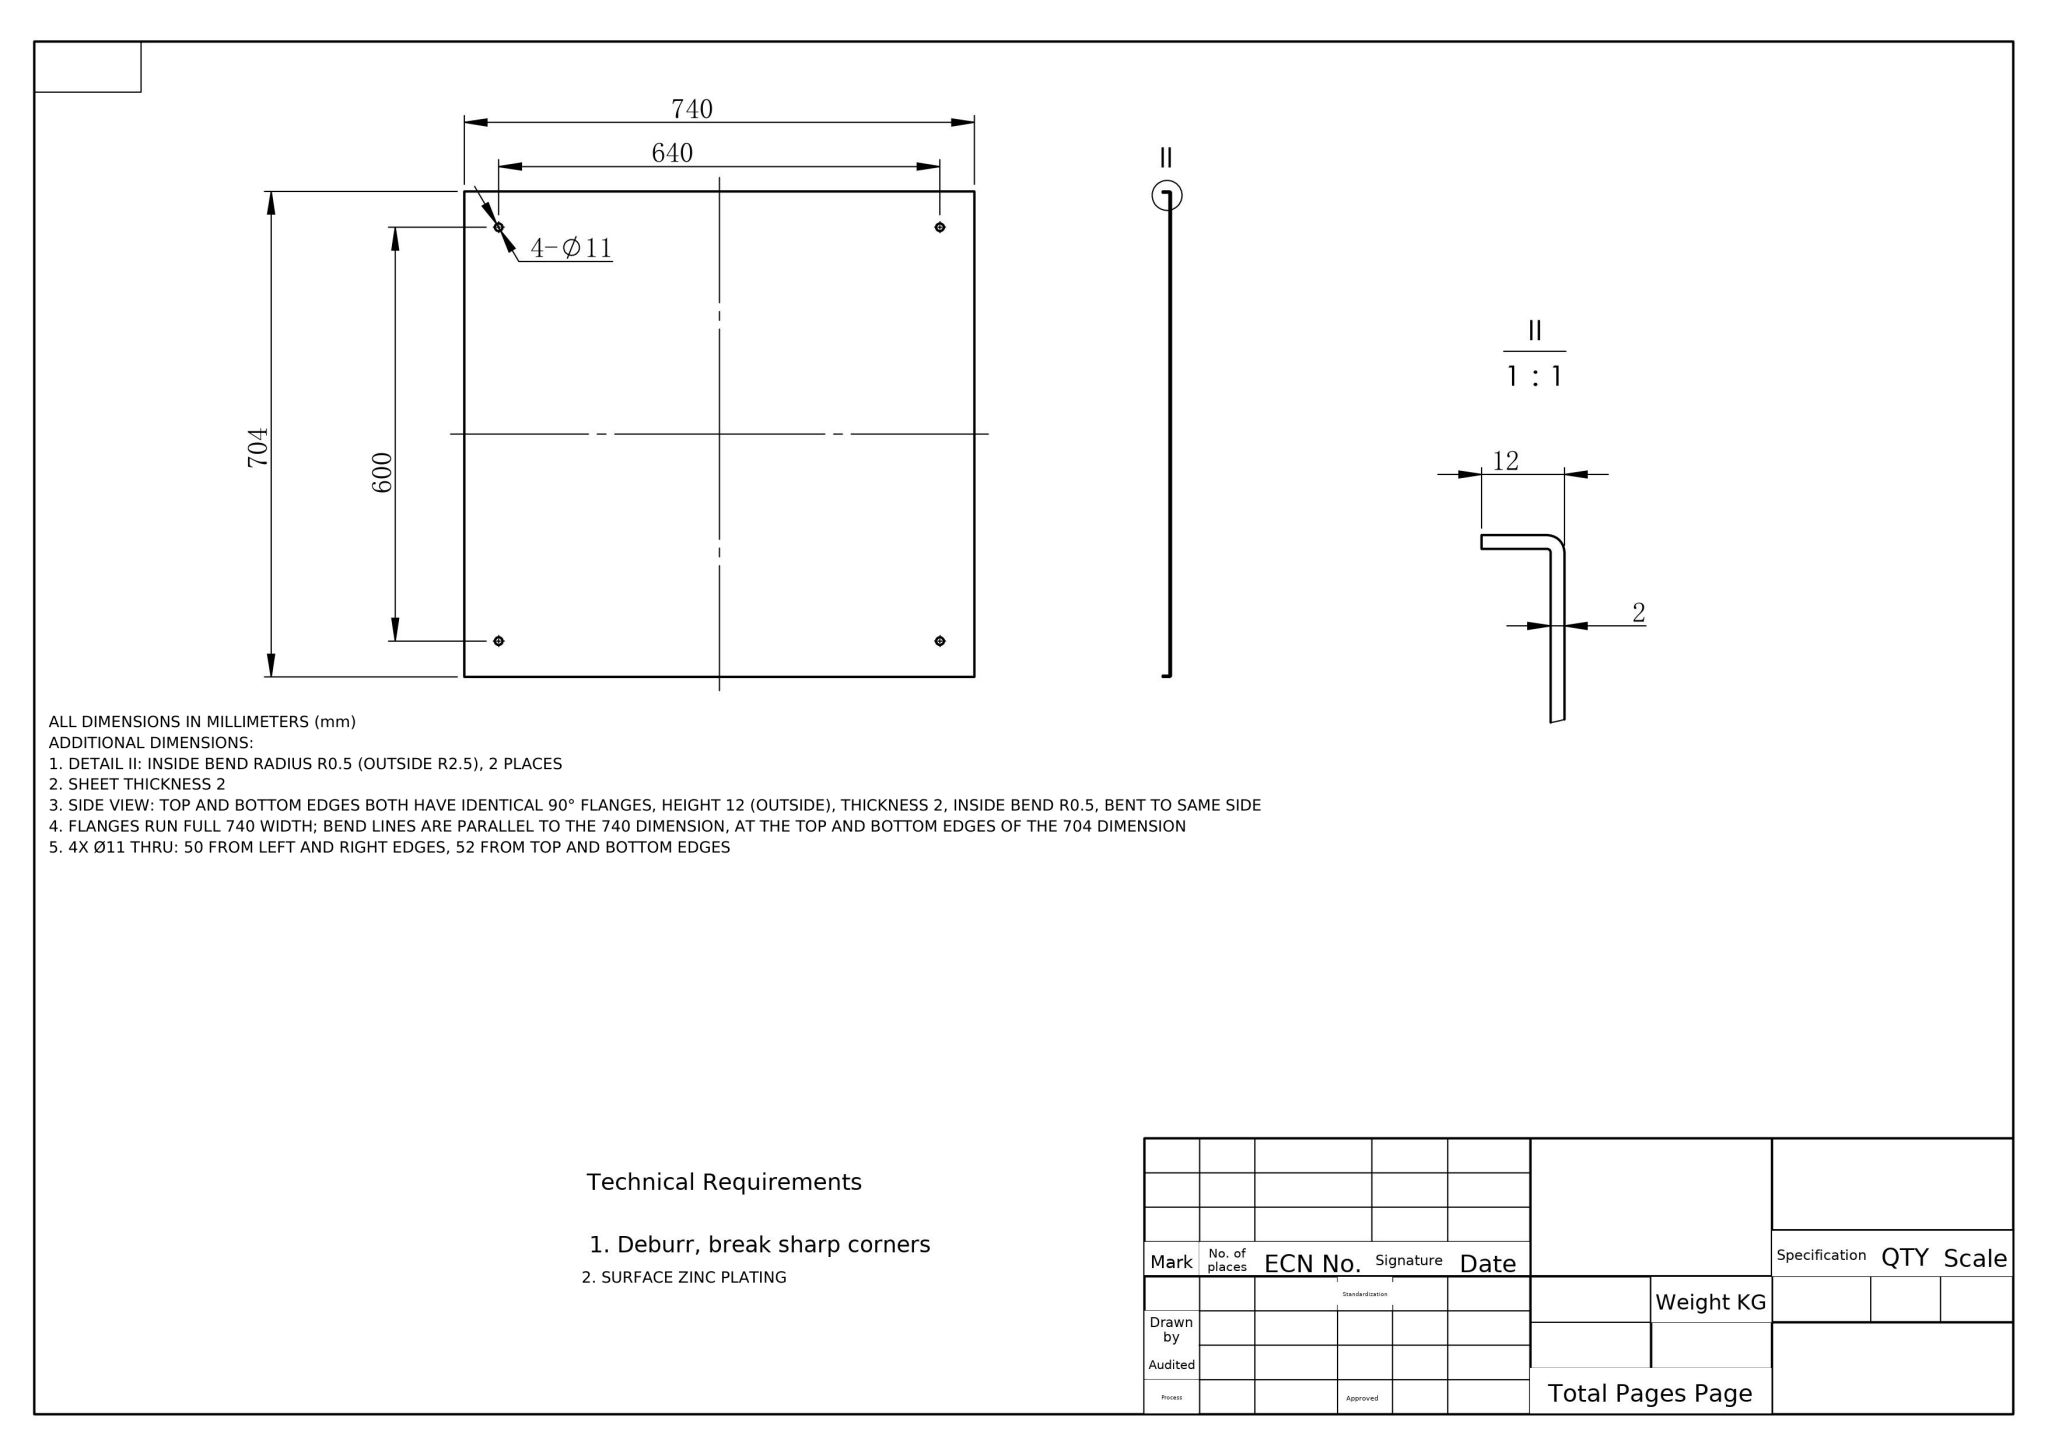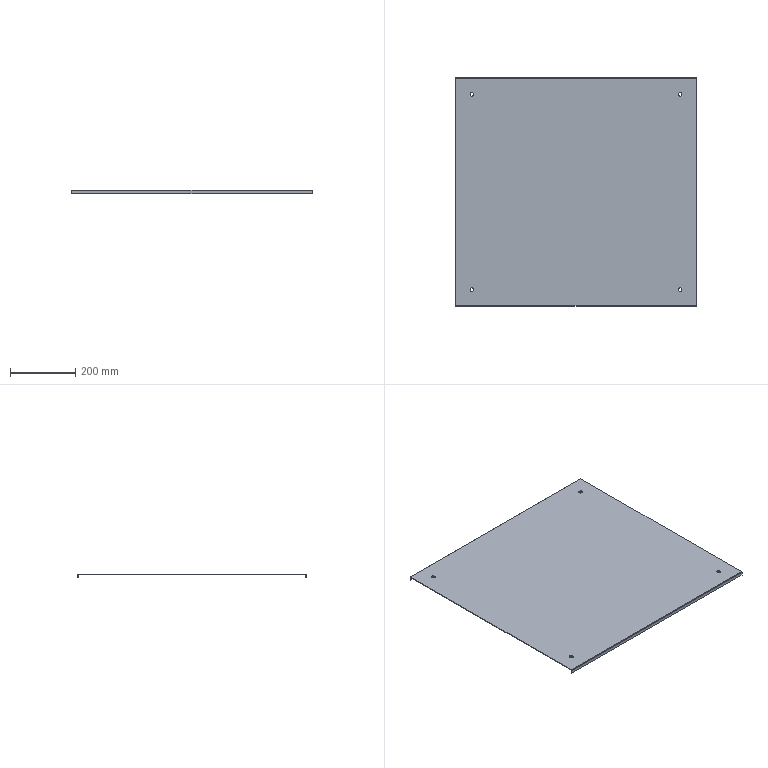Part | NX | mm | 1 solid | 30 faces | box 740 x 704 x 12 mm | volume 1068854 mm3 | plane 18 | cylinder 12 | commonest cylinder face diameters 11 x8 5 x2 1 x2
STEP:
#1=COLOUR_RGB('',0.5294,0.549,0.549);
#2=FILL_AREA_STYLE_COLOUR('',#1);
#3=FILL_AREA_STYLE('',(#2));
#4=SURFACE_STYLE_FILL_AREA(#3);
#5=SURFACE_SIDE_STYLE('',(#4));
#6=SURFACE_STYLE_USAGE(.BOTH.,#5);
#7=PRESENTATION_STYLE_ASSIGNMENT((#6));
#8=CARTESIAN_POINT('',(-305.5,600.,10.));
#9=VERTEX_POINT('',#8);
#10=CARTESIAN_POINT('',(-294.5,600.,10.));
#11=VERTEX_POINT('',#10);
#12=CARTESIAN_POINT('',(-300.,600.,10.));
#13=DIRECTION('',(0.,0.,1.));
#14=DIRECTION('',(1.,0.,0.));
#15=AXIS2_PLACEMENT_3D('',#12,#13,#14);
#16=CIRCLE('',#15,5.5);
#17=EDGE_CURVE('',#9,#11,#16,.T.);
#18=ORIENTED_EDGE('',*,*,#17,.F.);
#19=CARTESIAN_POINT('',(-305.5,600.,12.));
#20=VERTEX_POINT('',#19);
#21=CARTESIAN_POINT('',(-305.5,600.,12.));
#22=DIRECTION('',(0.,0.,1.));
#23=VECTOR('',#22,1000.);
#24=LINE('',#21,#23);
#25=EDGE_CURVE('',#9,#20,#24,.T.);
#26=ORIENTED_EDGE('',*,*,#25,.T.);
#27=CARTESIAN_POINT('',(-294.5,600.,12.));
#28=VERTEX_POINT('',#27);
#29=CARTESIAN_POINT('',(-300.,600.,12.));
#30=DIRECTION('',(0.,0.,1.));
#31=DIRECTION('',(-1.,0.,0.));
#32=AXIS2_PLACEMENT_3D('',#29,#30,#31);
#33=CIRCLE('',#32,5.5);
#34=EDGE_CURVE('',#20,#28,#33,.T.);
#35=ORIENTED_EDGE('',*,*,#34,.T.);
#36=CARTESIAN_POINT('',(-294.5,600.,12.));
#37=DIRECTION('',(0.,0.,1.));
#38=VECTOR('',#37,1000.);
#39=LINE('',#36,#38);
#40=EDGE_CURVE('',#11,#28,#39,.T.);
#41=ORIENTED_EDGE('',*,*,#40,.F.);
#42=EDGE_LOOP('',(#18,#26,#35,#41));
#43=FACE_OUTER_BOUND('',#42,.T.);
#44=CARTESIAN_POINT('',(-300.,600.,12.));
#45=DIRECTION('',(0.,0.,1.));
#46=DIRECTION('',(1.,0.,0.));
#47=AXIS2_PLACEMENT_3D('',#44,#45,#46);
#48=CYLINDRICAL_SURFACE('',#47,5.5);
#49=ADVANCED_FACE('',(#43),#48,.F.);
#50=CARTESIAN_POINT('',(334.5,600.,10.));
#51=VERTEX_POINT('',#50);
#52=CARTESIAN_POINT('',(345.5,600.,10.));
#53=VERTEX_POINT('',#52);
#54=CARTESIAN_POINT('',(340.,600.,10.));
#55=DIRECTION('',(0.,0.,1.));
#56=DIRECTION('',(1.,0.,0.));
#57=AXIS2_PLACEMENT_3D('',#54,#55,#56);
#58=CIRCLE('',#57,5.5);
#59=EDGE_CURVE('',#51,#53,#58,.T.);
#60=ORIENTED_EDGE('',*,*,#59,.F.);
#61=CARTESIAN_POINT('',(334.5,600.,12.));
#62=VERTEX_POINT('',#61);
#63=CARTESIAN_POINT('',(334.5,600.,12.));
#64=DIRECTION('',(0.,0.,1.));
#65=VECTOR('',#64,1000.);
#66=LINE('',#63,#65);
#67=EDGE_CURVE('',#51,#62,#66,.T.);
#68=ORIENTED_EDGE('',*,*,#67,.T.);
#69=CARTESIAN_POINT('',(345.5,600.,12.));
#70=VERTEX_POINT('',#69);
#71=CARTESIAN_POINT('',(340.,600.,12.));
#72=DIRECTION('',(0.,0.,1.));
#73=DIRECTION('',(-1.,0.,0.));
#74=AXIS2_PLACEMENT_3D('',#71,#72,#73);
#75=CIRCLE('',#74,5.5);
#76=EDGE_CURVE('',#62,#70,#75,.T.);
#77=ORIENTED_EDGE('',*,*,#76,.T.);
#78=CARTESIAN_POINT('',(345.5,600.,12.));
#79=DIRECTION('',(0.,0.,1.));
#80=VECTOR('',#79,1000.);
#81=LINE('',#78,#80);
#82=EDGE_CURVE('',#53,#70,#81,.T.);
#83=ORIENTED_EDGE('',*,*,#82,.F.);
#84=EDGE_LOOP('',(#60,#68,#77,#83));
#85=FACE_OUTER_BOUND('',#84,.T.);
#86=CARTESIAN_POINT('',(340.,600.,12.));
#87=DIRECTION('',(0.,0.,1.));
#88=DIRECTION('',(1.,0.,0.));
#89=AXIS2_PLACEMENT_3D('',#86,#87,#88);
#90=CYLINDRICAL_SURFACE('',#89,5.5);
#91=ADVANCED_FACE('',(#85),#90,.F.);
#92=CARTESIAN_POINT('',(334.5,1200.,10.));
#93=VERTEX_POINT('',#92);
#94=CARTESIAN_POINT('',(345.5,1200.,10.));
#95=VERTEX_POINT('',#94);
#96=CARTESIAN_POINT('',(340.,1200.,10.));
#97=DIRECTION('',(0.,0.,1.));
#98=DIRECTION('',(1.,0.,0.));
#99=AXIS2_PLACEMENT_3D('',#96,#97,#98);
#100=CIRCLE('',#99,5.5);
#101=EDGE_CURVE('',#93,#95,#100,.T.);
#102=ORIENTED_EDGE('',*,*,#101,.F.);
#103=CARTESIAN_POINT('',(334.5,1200.,12.));
#104=VERTEX_POINT('',#103);
#105=CARTESIAN_POINT('',(334.5,1200.,12.));
#106=DIRECTION('',(0.,0.,1.));
#107=VECTOR('',#106,1000.);
#108=LINE('',#105,#107);
#109=EDGE_CURVE('',#93,#104,#108,.T.);
#110=ORIENTED_EDGE('',*,*,#109,.T.);
#111=CARTESIAN_POINT('',(345.5,1200.,12.));
#112=VERTEX_POINT('',#111);
#113=CARTESIAN_POINT('',(340.,1200.,12.));
#114=DIRECTION('',(0.,0.,1.));
#115=DIRECTION('',(1.,0.,0.));
#116=AXIS2_PLACEMENT_3D('',#113,#114,#115);
#117=CIRCLE('',#116,5.5);
#118=EDGE_CURVE('',#104,#112,#117,.T.);
#119=ORIENTED_EDGE('',*,*,#118,.T.);
#120=CARTESIAN_POINT('',(345.5,1200.,12.));
#121=DIRECTION('',(0.,0.,1.));
#122=VECTOR('',#121,1000.);
#123=LINE('',#120,#122);
#124=EDGE_CURVE('',#95,#112,#123,.T.);
#125=ORIENTED_EDGE('',*,*,#124,.F.);
#126=EDGE_LOOP('',(#102,#110,#119,#125));
#127=FACE_OUTER_BOUND('',#126,.T.);
#128=CARTESIAN_POINT('',(340.,1200.,12.));
#129=DIRECTION('',(0.,0.,1.));
#130=DIRECTION('',(1.,0.,0.));
#131=AXIS2_PLACEMENT_3D('',#128,#129,#130);
#132=CYLINDRICAL_SURFACE('',#131,5.5);
#133=ADVANCED_FACE('',(#127),#132,.F.);
#134=CARTESIAN_POINT('',(-305.5,1200.,10.));
#135=VERTEX_POINT('',#134);
#136=CARTESIAN_POINT('',(-294.5,1200.,10.));
#137=VERTEX_POINT('',#136);
#138=CARTESIAN_POINT('',(-300.,1200.,10.));
#139=DIRECTION('',(0.,0.,1.));
#140=DIRECTION('',(1.,0.,0.));
#141=AXIS2_PLACEMENT_3D('',#138,#139,#140);
#142=CIRCLE('',#141,5.5);
#143=EDGE_CURVE('',#135,#137,#142,.T.);
#144=ORIENTED_EDGE('',*,*,#143,.F.);
#145=CARTESIAN_POINT('',(-305.5,1200.,12.));
#146=VERTEX_POINT('',#145);
#147=CARTESIAN_POINT('',(-305.5,1200.,12.));
#148=DIRECTION('',(0.,0.,1.));
#149=VECTOR('',#148,1000.);
#150=LINE('',#147,#149);
#151=EDGE_CURVE('',#135,#146,#150,.T.);
#152=ORIENTED_EDGE('',*,*,#151,.T.);
#153=CARTESIAN_POINT('',(-294.5,1200.,12.));
#154=VERTEX_POINT('',#153);
#155=CARTESIAN_POINT('',(-300.,1200.,12.));
#156=DIRECTION('',(0.,0.,1.));
#157=DIRECTION('',(1.,0.,0.));
#158=AXIS2_PLACEMENT_3D('',#155,#156,#157);
#159=CIRCLE('',#158,5.5);
#160=EDGE_CURVE('',#146,#154,#159,.T.);
#161=ORIENTED_EDGE('',*,*,#160,.T.);
#162=CARTESIAN_POINT('',(-294.5,1200.,12.));
#163=DIRECTION('',(0.,0.,1.));
#164=VECTOR('',#163,1000.);
#165=LINE('',#162,#164);
#166=EDGE_CURVE('',#137,#154,#165,.T.);
#167=ORIENTED_EDGE('',*,*,#166,.F.);
#168=EDGE_LOOP('',(#144,#152,#161,#167));
#169=FACE_OUTER_BOUND('',#168,.T.);
#170=CARTESIAN_POINT('',(-300.,1200.,12.));
#171=DIRECTION('',(0.,0.,1.));
#172=DIRECTION('',(1.,0.,0.));
#173=AXIS2_PLACEMENT_3D('',#170,#171,#172);
#174=CYLINDRICAL_SURFACE('',#173,5.5);
#175=ADVANCED_FACE('',(#169),#174,.F.);
#176=CARTESIAN_POINT('',(-300.,1200.,12.));
#177=DIRECTION('',(0.,0.,1.));
#178=DIRECTION('',(1.,0.,0.));
#179=AXIS2_PLACEMENT_3D('',#176,#177,#178);
#180=CIRCLE('',#179,5.5);
#181=EDGE_CURVE('',#154,#146,#180,.T.);
#182=ORIENTED_EDGE('',*,*,#181,.F.);
#183=ORIENTED_EDGE('',*,*,#160,.F.);
#184=EDGE_LOOP('',(#182,#183));
#185=FACE_BOUND('',#184,.T.);
#186=CARTESIAN_POINT('',(340.,1200.,12.));
#187=DIRECTION('',(0.,0.,1.));
#188=DIRECTION('',(1.,0.,0.));
#189=AXIS2_PLACEMENT_3D('',#186,#187,#188);
#190=CIRCLE('',#189,5.5);
#191=EDGE_CURVE('',#112,#104,#190,.T.);
#192=ORIENTED_EDGE('',*,*,#191,.F.);
#193=ORIENTED_EDGE('',*,*,#118,.F.);
#194=EDGE_LOOP('',(#192,#193));
#195=FACE_BOUND('',#194,.T.);
#196=CARTESIAN_POINT('',(340.,600.,12.));
#197=DIRECTION('',(0.,0.,1.));
#198=DIRECTION('',(-1.,0.,0.));
#199=AXIS2_PLACEMENT_3D('',#196,#197,#198);
#200=CIRCLE('',#199,5.5);
#201=EDGE_CURVE('',#70,#62,#200,.T.);
#202=ORIENTED_EDGE('',*,*,#201,.F.);
#203=ORIENTED_EDGE('',*,*,#76,.F.);
#204=EDGE_LOOP('',(#202,#203));
#205=FACE_BOUND('',#204,.T.);
#206=CARTESIAN_POINT('',(-300.,600.,12.));
#207=DIRECTION('',(0.,0.,1.));
#208=DIRECTION('',(-1.,0.,0.));
#209=AXIS2_PLACEMENT_3D('',#206,#207,#208);
#210=CIRCLE('',#209,5.5);
#211=EDGE_CURVE('',#28,#20,#210,.T.);
#212=ORIENTED_EDGE('',*,*,#211,.F.);
#213=ORIENTED_EDGE('',*,*,#34,.F.);
#214=EDGE_LOOP('',(#212,#213));
#215=FACE_BOUND('',#214,.T.);
#216=CARTESIAN_POINT('',(-350.,550.5,12.));
#217=VERTEX_POINT('',#216);
#218=CARTESIAN_POINT('',(390.,550.5,12.));
#219=VERTEX_POINT('',#218);
#220=CARTESIAN_POINT('',(-350.,550.5,12.));
#221=DIRECTION('',(1.,0.,0.));
#222=VECTOR('',#221,1000.);
#223=LINE('',#220,#222);
#224=EDGE_CURVE('',#217,#219,#223,.T.);
#225=ORIENTED_EDGE('',*,*,#224,.T.);
#226=CARTESIAN_POINT('',(390.,1249.5,12.));
#227=VERTEX_POINT('',#226);
#228=CARTESIAN_POINT('',(390.,550.,12.));
#229=DIRECTION('',(0.,1.,0.));
#230=VECTOR('',#229,1000.);
#231=LINE('',#228,#230);
#232=EDGE_CURVE('',#219,#227,#231,.T.);
#233=ORIENTED_EDGE('',*,*,#232,.T.);
#234=CARTESIAN_POINT('',(-350.,1249.5,12.));
#235=VERTEX_POINT('',#234);
#236=CARTESIAN_POINT('',(390.,1249.5,12.));
#237=DIRECTION('',(-1.,0.,0.));
#238=VECTOR('',#237,1000.);
#239=LINE('',#236,#238);
#240=EDGE_CURVE('',#227,#235,#239,.T.);
#241=ORIENTED_EDGE('',*,*,#240,.T.);
#242=CARTESIAN_POINT('',(-350.,550.,12.));
#243=DIRECTION('',(0.,-1.,0.));
#244=VECTOR('',#243,1000.);
#245=LINE('',#242,#244);
#246=EDGE_CURVE('',#235,#217,#245,.T.);
#247=ORIENTED_EDGE('',*,*,#246,.T.);
#248=EDGE_LOOP('',(#225,#233,#241,#247));
#249=FACE_OUTER_BOUND('',#248,.T.);
#250=CARTESIAN_POINT('',(0.,0.,12.));
#251=DIRECTION('',(0.,0.,-1.));
#252=DIRECTION('',(-1.,0.,0.));
#253=AXIS2_PLACEMENT_3D('',#250,#251,#252);
#254=PLANE('',#253);
#255=ADVANCED_FACE('',(#185,#195,#205,#215,#249),#254,.F.);
#256=CARTESIAN_POINT('',(-300.,1200.,10.));
#257=DIRECTION('',(0.,0.,1.));
#258=DIRECTION('',(1.,0.,0.));
#259=AXIS2_PLACEMENT_3D('',#256,#257,#258);
#260=CIRCLE('',#259,5.5);
#261=EDGE_CURVE('',#137,#135,#260,.T.);
#262=ORIENTED_EDGE('',*,*,#261,.T.);
#263=ORIENTED_EDGE('',*,*,#143,.T.);
#264=EDGE_LOOP('',(#262,#263));
#265=FACE_BOUND('',#264,.T.);
#266=CARTESIAN_POINT('',(340.,1200.,10.));
#267=DIRECTION('',(0.,0.,1.));
#268=DIRECTION('',(1.,0.,0.));
#269=AXIS2_PLACEMENT_3D('',#266,#267,#268);
#270=CIRCLE('',#269,5.5);
#271=EDGE_CURVE('',#95,#93,#270,.T.);
#272=ORIENTED_EDGE('',*,*,#271,.T.);
#273=ORIENTED_EDGE('',*,*,#101,.T.);
#274=EDGE_LOOP('',(#272,#273));
#275=FACE_BOUND('',#274,.T.);
#276=CARTESIAN_POINT('',(340.,600.,10.));
#277=DIRECTION('',(0.,0.,1.));
#278=DIRECTION('',(1.,0.,0.));
#279=AXIS2_PLACEMENT_3D('',#276,#277,#278);
#280=CIRCLE('',#279,5.5);
#281=EDGE_CURVE('',#53,#51,#280,.T.);
#282=ORIENTED_EDGE('',*,*,#281,.T.);
#283=ORIENTED_EDGE('',*,*,#59,.T.);
#284=EDGE_LOOP('',(#282,#283));
#285=FACE_BOUND('',#284,.T.);
#286=CARTESIAN_POINT('',(-300.,600.,10.));
#287=DIRECTION('',(0.,0.,1.));
#288=DIRECTION('',(1.,0.,0.));
#289=AXIS2_PLACEMENT_3D('',#286,#287,#288);
#290=CIRCLE('',#289,5.5);
#291=EDGE_CURVE('',#11,#9,#290,.T.);
#292=ORIENTED_EDGE('',*,*,#291,.T.);
#293=ORIENTED_EDGE('',*,*,#17,.T.);
#294=EDGE_LOOP('',(#292,#293));
#295=FACE_BOUND('',#294,.T.);
#296=CARTESIAN_POINT('',(390.,550.5,10.));
#297=VERTEX_POINT('',#296);
#298=CARTESIAN_POINT('',(390.,1249.5,10.));
#299=VERTEX_POINT('',#298);
#300=CARTESIAN_POINT('',(390.,0.,10.));
#301=DIRECTION('',(0.,1.,0.));
#302=VECTOR('',#301,1000.);
#303=LINE('',#300,#302);
#304=EDGE_CURVE('',#297,#299,#303,.T.);
#305=ORIENTED_EDGE('',*,*,#304,.F.);
#306=CARTESIAN_POINT('',(-350.,550.5,10.));
#307=VERTEX_POINT('',#306);
#308=CARTESIAN_POINT('',(-350.,550.5,10.));
#309=DIRECTION('',(1.,0.,0.));
#310=VECTOR('',#309,1000.);
#311=LINE('',#308,#310);
#312=EDGE_CURVE('',#307,#297,#311,.T.);
#313=ORIENTED_EDGE('',*,*,#312,.F.);
#314=CARTESIAN_POINT('',(-350.,1249.5,10.));
#315=VERTEX_POINT('',#314);
#316=CARTESIAN_POINT('',(-350.,0.,10.));
#317=DIRECTION('',(0.,-1.,0.));
#318=VECTOR('',#317,1000.);
#319=LINE('',#316,#318);
#320=EDGE_CURVE('',#315,#307,#319,.T.);
#321=ORIENTED_EDGE('',*,*,#320,.F.);
#322=CARTESIAN_POINT('',(390.,1249.5,10.));
#323=DIRECTION('',(-1.,0.,0.));
#324=VECTOR('',#323,1000.);
#325=LINE('',#322,#324);
#326=EDGE_CURVE('',#299,#315,#325,.T.);
#327=ORIENTED_EDGE('',*,*,#326,.F.);
#328=EDGE_LOOP('',(#305,#313,#321,#327));
#329=FACE_OUTER_BOUND('',#328,.T.);
#330=CARTESIAN_POINT('',(0.,0.,10.));
#331=DIRECTION('',(0.,0.,-1.));
#332=DIRECTION('',(-1.,0.,0.));
#333=AXIS2_PLACEMENT_3D('',#330,#331,#332);
#334=PLANE('',#333);
#335=ADVANCED_FACE('',(#265,#275,#285,#295,#329),#334,.T.);
#336=ORIENTED_EDGE('',*,*,#320,.T.);
#337=CARTESIAN_POINT('',(-350.,550.5,10.));
#338=DIRECTION('',(0.,0.,1.));
#339=VECTOR('',#338,1000.);
#340=LINE('',#337,#339);
#341=EDGE_CURVE('',#307,#217,#340,.T.);
#342=ORIENTED_EDGE('',*,*,#341,.T.);
#343=ORIENTED_EDGE('',*,*,#246,.F.);
#344=CARTESIAN_POINT('',(-350.,1249.5,10.));
#345=DIRECTION('',(0.,0.,1.));
#346=VECTOR('',#345,1000.);
#347=LINE('',#344,#346);
#348=EDGE_CURVE('',#315,#235,#347,.T.);
#349=ORIENTED_EDGE('',*,*,#348,.F.);
#350=EDGE_LOOP('',(#336,#342,#343,#349));
#351=FACE_OUTER_BOUND('',#350,.T.);
#352=CARTESIAN_POINT('',(-350.,550.,12.));
#353=DIRECTION('',(1.,0.,0.));
#354=DIRECTION('',(0.,-1.,0.));
#355=AXIS2_PLACEMENT_3D('',#352,#353,#354);
#356=PLANE('',#355);
#357=ADVANCED_FACE('',(#351),#356,.F.);
#358=CARTESIAN_POINT('',(390.,550.5,10.));
#359=DIRECTION('',(0.,0.,1.));
#360=VECTOR('',#359,1000.);
#361=LINE('',#358,#360);
#362=EDGE_CURVE('',#297,#219,#361,.T.);
#363=ORIENTED_EDGE('',*,*,#362,.F.);
#364=ORIENTED_EDGE('',*,*,#304,.T.);
#365=CARTESIAN_POINT('',(390.,1249.5,10.));
#366=DIRECTION('',(0.,0.,1.));
#367=VECTOR('',#366,1000.);
#368=LINE('',#365,#367);
#369=EDGE_CURVE('',#299,#227,#368,.T.);
#370=ORIENTED_EDGE('',*,*,#369,.T.);
#371=ORIENTED_EDGE('',*,*,#232,.F.);
#372=EDGE_LOOP('',(#363,#364,#370,#371));
#373=FACE_OUTER_BOUND('',#372,.T.);
#374=CARTESIAN_POINT('',(390.,550.,12.));
#375=DIRECTION('',(-1.,0.,0.));
#376=DIRECTION('',(0.,1.,0.));
#377=AXIS2_PLACEMENT_3D('',#374,#375,#376);
#378=PLANE('',#377);
#379=ADVANCED_FACE('',(#373),#378,.F.);
#380=ORIENTED_EDGE('',*,*,#151,.F.);
#381=ORIENTED_EDGE('',*,*,#261,.F.);
#382=ORIENTED_EDGE('',*,*,#166,.T.);
#383=ORIENTED_EDGE('',*,*,#181,.T.);
#384=EDGE_LOOP('',(#380,#381,#382,#383));
#385=FACE_OUTER_BOUND('',#384,.T.);
#386=CARTESIAN_POINT('',(-300.,1200.,12.));
#387=DIRECTION('',(0.,0.,1.));
#388=DIRECTION('',(1.,0.,0.));
#389=AXIS2_PLACEMENT_3D('',#386,#387,#388);
#390=CYLINDRICAL_SURFACE('',#389,5.5);
#391=ADVANCED_FACE('',(#385),#390,.F.);
#392=ORIENTED_EDGE('',*,*,#109,.F.);
#393=ORIENTED_EDGE('',*,*,#271,.F.);
#394=ORIENTED_EDGE('',*,*,#124,.T.);
#395=ORIENTED_EDGE('',*,*,#191,.T.);
#396=EDGE_LOOP('',(#392,#393,#394,#395));
#397=FACE_OUTER_BOUND('',#396,.T.);
#398=CARTESIAN_POINT('',(340.,1200.,12.));
#399=DIRECTION('',(0.,0.,1.));
#400=DIRECTION('',(1.,0.,0.));
#401=AXIS2_PLACEMENT_3D('',#398,#399,#400);
#402=CYLINDRICAL_SURFACE('',#401,5.5);
#403=ADVANCED_FACE('',(#397),#402,.F.);
#404=ORIENTED_EDGE('',*,*,#67,.F.);
#405=ORIENTED_EDGE('',*,*,#281,.F.);
#406=ORIENTED_EDGE('',*,*,#82,.T.);
#407=ORIENTED_EDGE('',*,*,#201,.T.);
#408=EDGE_LOOP('',(#404,#405,#406,#407));
#409=FACE_OUTER_BOUND('',#408,.T.);
#410=CARTESIAN_POINT('',(340.,600.,12.));
#411=DIRECTION('',(0.,0.,1.));
#412=DIRECTION('',(1.,0.,0.));
#413=AXIS2_PLACEMENT_3D('',#410,#411,#412);
#414=CYLINDRICAL_SURFACE('',#413,5.5);
#415=ADVANCED_FACE('',(#409),#414,.F.);
#416=ORIENTED_EDGE('',*,*,#25,.F.);
#417=ORIENTED_EDGE('',*,*,#291,.F.);
#418=ORIENTED_EDGE('',*,*,#40,.T.);
#419=ORIENTED_EDGE('',*,*,#211,.T.);
#420=EDGE_LOOP('',(#416,#417,#418,#419));
#421=FACE_OUTER_BOUND('',#420,.T.);
#422=CARTESIAN_POINT('',(-300.,600.,12.));
#423=DIRECTION('',(0.,0.,1.));
#424=DIRECTION('',(1.,0.,0.));
#425=AXIS2_PLACEMENT_3D('',#422,#423,#424);
#426=CYLINDRICAL_SURFACE('',#425,5.5);
#427=ADVANCED_FACE('',(#421),#426,.F.);
#428=CARTESIAN_POINT('',(-350.,1250.,9.5));
#429=VERTEX_POINT('',#428);
#430=CARTESIAN_POINT('',(-350.,1252.,9.5));
#431=VERTEX_POINT('',#430);
#432=CARTESIAN_POINT('',(-350.,1250.,9.5));
#433=DIRECTION('',(0.,1.,0.));
#434=VECTOR('',#433,1000.);
#435=LINE('',#432,#434);
#436=EDGE_CURVE('',#429,#431,#435,.T.);
#437=ORIENTED_EDGE('',*,*,#436,.F.);
#438=CARTESIAN_POINT('',(-350.,1249.5,9.5));
#439=DIRECTION('',(-1.,0.,0.));
#440=DIRECTION('',(0.,0.,-1.));
#441=AXIS2_PLACEMENT_3D('',#438,#439,#440);
#442=CIRCLE('',#441,0.5);
#443=EDGE_CURVE('',#315,#429,#442,.T.);
#444=ORIENTED_EDGE('',*,*,#443,.F.);
#445=ORIENTED_EDGE('',*,*,#348,.T.);
#446=CARTESIAN_POINT('',(-350.,1249.5,9.5));
#447=DIRECTION('',(-1.,0.,0.));
#448=DIRECTION('',(0.,0.,-1.));
#449=AXIS2_PLACEMENT_3D('',#446,#447,#448);
#450=CIRCLE('',#449,2.5);
#451=EDGE_CURVE('',#235,#431,#450,.T.);
#452=ORIENTED_EDGE('',*,*,#451,.T.);
#453=EDGE_LOOP('',(#437,#444,#445,#452));
#454=FACE_OUTER_BOUND('',#453,.T.);
#455=CARTESIAN_POINT('',(-350.,1249.5,9.5));
#456=DIRECTION('',(-1.,0.,0.));
#457=DIRECTION('',(0.,0.,1.));
#458=AXIS2_PLACEMENT_3D('',#455,#456,#457);
#459=PLANE('',#458);
#460=ADVANCED_FACE('',(#454),#459,.T.);
#461=CARTESIAN_POINT('',(390.,1250.,9.5));
#462=VERTEX_POINT('',#461);
#463=CARTESIAN_POINT('',(390.,1249.5,9.5));
#464=DIRECTION('',(1.,0.,0.));
#465=DIRECTION('',(0.,0.,-1.));
#466=AXIS2_PLACEMENT_3D('',#463,#464,#465);
#467=CIRCLE('',#466,0.5);
#468=EDGE_CURVE('',#462,#299,#467,.T.);
#469=ORIENTED_EDGE('',*,*,#468,.F.);
#470=CARTESIAN_POINT('',(390.,1252.,9.5));
#471=VERTEX_POINT('',#470);
#472=CARTESIAN_POINT('',(390.,1250.,9.5));
#473=DIRECTION('',(0.,1.,0.));
#474=VECTOR('',#473,1000.);
#475=LINE('',#472,#474);
#476=EDGE_CURVE('',#462,#471,#475,.T.);
#477=ORIENTED_EDGE('',*,*,#476,.T.);
#478=CARTESIAN_POINT('',(390.,1249.5,9.5));
#479=DIRECTION('',(1.,0.,0.));
#480=DIRECTION('',(0.,0.,-1.));
#481=AXIS2_PLACEMENT_3D('',#478,#479,#480);
#482=CIRCLE('',#481,2.5);
#483=EDGE_CURVE('',#471,#227,#482,.T.);
#484=ORIENTED_EDGE('',*,*,#483,.T.);
#485=ORIENTED_EDGE('',*,*,#369,.F.);
#486=EDGE_LOOP('',(#469,#477,#484,#485));
#487=FACE_OUTER_BOUND('',#486,.T.);
#488=CARTESIAN_POINT('',(390.,1249.5,9.5));
#489=DIRECTION('',(-1.,0.,0.));
#490=DIRECTION('',(0.,0.,1.));
#491=AXIS2_PLACEMENT_3D('',#488,#489,#490);
#492=PLANE('',#491);
#493=ADVANCED_FACE('',(#487),#492,.F.);
#494=ORIENTED_EDGE('',*,*,#240,.F.);
#495=ORIENTED_EDGE('',*,*,#483,.F.);
#496=CARTESIAN_POINT('',(0.,1252.,9.5));
#497=DIRECTION('',(-1.,0.,0.));
#498=VECTOR('',#497,1000.);
#499=LINE('',#496,#498);
#500=EDGE_CURVE('',#471,#431,#499,.T.);
#501=ORIENTED_EDGE('',*,*,#500,.T.);
#502=ORIENTED_EDGE('',*,*,#451,.F.);
#503=EDGE_LOOP('',(#494,#495,#501,#502));
#504=FACE_OUTER_BOUND('',#503,.T.);
#505=CARTESIAN_POINT('',(390.,1249.5,9.5));
#506=DIRECTION('',(1.,0.,0.));
#507=DIRECTION('',(0.,1.,0.));
#508=AXIS2_PLACEMENT_3D('',#505,#506,#507);
#509=CYLINDRICAL_SURFACE('',#508,2.5);
#510=ADVANCED_FACE('',(#504),#509,.T.);
#511=ORIENTED_EDGE('',*,*,#326,.T.);
#512=ORIENTED_EDGE('',*,*,#443,.T.);
#513=CARTESIAN_POINT('',(-350.,1250.,9.5));
#514=DIRECTION('',(1.,0.,0.));
#515=VECTOR('',#514,1000.);
#516=LINE('',#513,#515);
#517=EDGE_CURVE('',#429,#462,#516,.T.);
#518=ORIENTED_EDGE('',*,*,#517,.T.);
#519=ORIENTED_EDGE('',*,*,#468,.T.);
#520=EDGE_LOOP('',(#511,#512,#518,#519));
#521=FACE_OUTER_BOUND('',#520,.T.);
#522=CARTESIAN_POINT('',(390.,1249.5,9.5));
#523=DIRECTION('',(1.,0.,0.));
#524=DIRECTION('',(0.,1.,0.));
#525=AXIS2_PLACEMENT_3D('',#522,#523,#524);
#526=CYLINDRICAL_SURFACE('',#525,0.5);
#527=ADVANCED_FACE('',(#521),#526,.F.);
#528=CARTESIAN_POINT('',(-350.,1250.,0.));
#529=VERTEX_POINT('',#528);
#530=CARTESIAN_POINT('',(-350.,1250.,10.));
#531=DIRECTION('',(0.,0.,-1.));
#532=VECTOR('',#531,1000.);
#533=LINE('',#530,#532);
#534=EDGE_CURVE('',#429,#529,#533,.T.);
#535=ORIENTED_EDGE('',*,*,#534,.F.);
#536=ORIENTED_EDGE('',*,*,#436,.T.);
#537=CARTESIAN_POINT('',(-350.,1252.,0.));
#538=VERTEX_POINT('',#537);
#539=CARTESIAN_POINT('',(-350.,1252.,10.));
#540=DIRECTION('',(0.,0.,-1.));
#541=VECTOR('',#540,1000.);
#542=LINE('',#539,#541);
#543=EDGE_CURVE('',#431,#538,#542,.T.);
#544=ORIENTED_EDGE('',*,*,#543,.T.);
#545=CARTESIAN_POINT('',(-350.,1252.,0.));
#546=DIRECTION('',(0.,-1.,-0.));
#547=VECTOR('',#546,1000.);
#548=LINE('',#545,#547);
#549=EDGE_CURVE('',#538,#529,#548,.T.);
#550=ORIENTED_EDGE('',*,*,#549,.T.);
#551=EDGE_LOOP('',(#535,#536,#544,#550));
#552=FACE_OUTER_BOUND('',#551,.T.);
#553=CARTESIAN_POINT('',(-350.,1252.,10.));
#554=DIRECTION('',(-1.,0.,0.));
#555=DIRECTION('',(0.,0.,1.));
#556=AXIS2_PLACEMENT_3D('',#553,#554,#555);
#557=PLANE('',#556);
#558=ADVANCED_FACE('',(#552),#557,.T.);
#559=CARTESIAN_POINT('',(390.,1252.,0.));
#560=VERTEX_POINT('',#559);
#561=CARTESIAN_POINT('',(390.,1252.,0.));
#562=DIRECTION('',(0.,0.,1.));
#563=VECTOR('',#562,1000.);
#564=LINE('',#561,#563);
#565=EDGE_CURVE('',#560,#471,#564,.T.);
#566=ORIENTED_EDGE('',*,*,#565,.T.);
#567=ORIENTED_EDGE('',*,*,#476,.F.);
#568=CARTESIAN_POINT('',(390.,1250.,0.));
#569=VERTEX_POINT('',#568);
#570=CARTESIAN_POINT('',(390.,1250.,0.));
#571=DIRECTION('',(0.,0.,1.));
#572=VECTOR('',#571,1000.);
#573=LINE('',#570,#572);
#574=EDGE_CURVE('',#569,#462,#573,.T.);
#575=ORIENTED_EDGE('',*,*,#574,.F.);
#576=CARTESIAN_POINT('',(390.,1252.,0.));
#577=DIRECTION('',(0.,-1.,-0.));
#578=VECTOR('',#577,1000.);
#579=LINE('',#576,#578);
#580=EDGE_CURVE('',#560,#569,#579,.T.);
#581=ORIENTED_EDGE('',*,*,#580,.F.);
#582=EDGE_LOOP('',(#566,#567,#575,#581));
#583=FACE_OUTER_BOUND('',#582,.T.);
#584=CARTESIAN_POINT('',(390.,1252.,0.));
#585=DIRECTION('',(1.,0.,0.));
#586=DIRECTION('',(0.,0.,-1.));
#587=AXIS2_PLACEMENT_3D('',#584,#585,#586);
#588=PLANE('',#587);
#589=ADVANCED_FACE('',(#583),#588,.T.);
#590=ORIENTED_EDGE('',*,*,#500,.F.);
#591=ORIENTED_EDGE('',*,*,#565,.F.);
#592=CARTESIAN_POINT('',(-350.,1252.,0.));
#593=DIRECTION('',(1.,0.,0.));
#594=VECTOR('',#593,1000.);
#595=LINE('',#592,#594);
#596=EDGE_CURVE('',#538,#560,#595,.T.);
#597=ORIENTED_EDGE('',*,*,#596,.F.);
#598=ORIENTED_EDGE('',*,*,#543,.F.);
#599=EDGE_LOOP('',(#590,#591,#597,#598));
#600=FACE_OUTER_BOUND('',#599,.T.);
#601=CARTESIAN_POINT('',(0.,1252.,0.));
#602=DIRECTION('',(0.,-1.,0.));
#603=DIRECTION('',(0.,0.,-1.));
#604=AXIS2_PLACEMENT_3D('',#601,#602,#603);
#605=PLANE('',#604);
#606=ADVANCED_FACE('',(#600),#605,.F.);
#607=ORIENTED_EDGE('',*,*,#574,.T.);
#608=ORIENTED_EDGE('',*,*,#517,.F.);
#609=ORIENTED_EDGE('',*,*,#534,.T.);
#610=CARTESIAN_POINT('',(-350.,1250.,0.));
#611=DIRECTION('',(1.,0.,0.));
#612=VECTOR('',#611,1000.);
#613=LINE('',#610,#612);
#614=EDGE_CURVE('',#529,#569,#613,.T.);
#615=ORIENTED_EDGE('',*,*,#614,.T.);
#616=EDGE_LOOP('',(#607,#608,#609,#615));
#617=FACE_OUTER_BOUND('',#616,.T.);
#618=CARTESIAN_POINT('',(0.,1250.,0.));
#619=DIRECTION('',(0.,-1.,0.));
#620=DIRECTION('',(0.,0.,-1.));
#621=AXIS2_PLACEMENT_3D('',#618,#619,#620);
#622=PLANE('',#621);
#623=ADVANCED_FACE('',(#617),#622,.T.);
#624=ORIENTED_EDGE('',*,*,#614,.F.);
#625=ORIENTED_EDGE('',*,*,#549,.F.);
#626=ORIENTED_EDGE('',*,*,#596,.T.);
#627=ORIENTED_EDGE('',*,*,#580,.T.);
#628=EDGE_LOOP('',(#624,#625,#626,#627));
#629=FACE_OUTER_BOUND('',#628,.T.);
#630=CARTESIAN_POINT('',(-350.,1252.,0.));
#631=DIRECTION('',(0.,0.,-1.));
#632=DIRECTION('',(0.,1.,0.));
#633=AXIS2_PLACEMENT_3D('',#630,#631,#632);
#634=PLANE('',#633);
#635=ADVANCED_FACE('',(#629),#634,.T.);
#636=CARTESIAN_POINT('',(390.,550.,9.5));
#637=VERTEX_POINT('',#636);
#638=CARTESIAN_POINT('',(390.,548.,9.5));
#639=VERTEX_POINT('',#638);
#640=CARTESIAN_POINT('',(390.,550.,9.5));
#641=DIRECTION('',(0.,-1.,0.));
#642=VECTOR('',#641,1000.);
#643=LINE('',#640,#642);
#644=EDGE_CURVE('',#637,#639,#643,.T.);
#645=ORIENTED_EDGE('',*,*,#644,.F.);
#646=CARTESIAN_POINT('',(390.,550.5,9.5));
#647=DIRECTION('',(1.,0.,0.));
#648=DIRECTION('',(0.,0.,1.));
#649=AXIS2_PLACEMENT_3D('',#646,#647,#648);
#650=CIRCLE('',#649,0.5);
#651=EDGE_CURVE('',#297,#637,#650,.T.);
#652=ORIENTED_EDGE('',*,*,#651,.F.);
#653=ORIENTED_EDGE('',*,*,#362,.T.);
#654=CARTESIAN_POINT('',(390.,550.5,9.5));
#655=DIRECTION('',(1.,0.,0.));
#656=DIRECTION('',(0.,0.,1.));
#657=AXIS2_PLACEMENT_3D('',#654,#655,#656);
#658=CIRCLE('',#657,2.5);
#659=EDGE_CURVE('',#219,#639,#658,.T.);
#660=ORIENTED_EDGE('',*,*,#659,.T.);
#661=EDGE_LOOP('',(#645,#652,#653,#660));
#662=FACE_OUTER_BOUND('',#661,.T.);
#663=CARTESIAN_POINT('',(390.,550.5,9.5));
#664=DIRECTION('',(1.,0.,0.));
#665=DIRECTION('',(0.,0.,-1.));
#666=AXIS2_PLACEMENT_3D('',#663,#664,#665);
#667=PLANE('',#666);
#668=ADVANCED_FACE('',(#662),#667,.T.);
#669=CARTESIAN_POINT('',(-350.,550.,9.5));
#670=VERTEX_POINT('',#669);
#671=CARTESIAN_POINT('',(-350.,550.5,9.5));
#672=DIRECTION('',(-1.,0.,0.));
#673=DIRECTION('',(0.,0.,1.));
#674=AXIS2_PLACEMENT_3D('',#671,#672,#673);
#675=CIRCLE('',#674,0.5);
#676=EDGE_CURVE('',#670,#307,#675,.T.);
#677=ORIENTED_EDGE('',*,*,#676,.F.);
#678=CARTESIAN_POINT('',(-350.,548.,9.5));
#679=VERTEX_POINT('',#678);
#680=CARTESIAN_POINT('',(-350.,550.,9.5));
#681=DIRECTION('',(0.,-1.,0.));
#682=VECTOR('',#681,1000.);
#683=LINE('',#680,#682);
#684=EDGE_CURVE('',#670,#679,#683,.T.);
#685=ORIENTED_EDGE('',*,*,#684,.T.);
#686=CARTESIAN_POINT('',(-350.,550.5,9.5));
#687=DIRECTION('',(-1.,0.,0.));
#688=DIRECTION('',(0.,0.,1.));
#689=AXIS2_PLACEMENT_3D('',#686,#687,#688);
#690=CIRCLE('',#689,2.5);
#691=EDGE_CURVE('',#679,#217,#690,.T.);
#692=ORIENTED_EDGE('',*,*,#691,.T.);
#693=ORIENTED_EDGE('',*,*,#341,.F.);
#694=EDGE_LOOP('',(#677,#685,#692,#693));
#695=FACE_OUTER_BOUND('',#694,.T.);
#696=CARTESIAN_POINT('',(-350.,550.5,9.5));
#697=DIRECTION('',(1.,0.,0.));
#698=DIRECTION('',(0.,0.,-1.));
#699=AXIS2_PLACEMENT_3D('',#696,#697,#698);
#700=PLANE('',#699);
#701=ADVANCED_FACE('',(#695),#700,.F.);
#702=ORIENTED_EDGE('',*,*,#224,.F.);
#703=ORIENTED_EDGE('',*,*,#691,.F.);
#704=CARTESIAN_POINT('',(0.,548.,9.5));
#705=DIRECTION('',(-1.,0.,0.));
#706=VECTOR('',#705,1000.);
#707=LINE('',#704,#706);
#708=EDGE_CURVE('',#639,#679,#707,.T.);
#709=ORIENTED_EDGE('',*,*,#708,.F.);
#710=ORIENTED_EDGE('',*,*,#659,.F.);
#711=EDGE_LOOP('',(#702,#703,#709,#710));
#712=FACE_OUTER_BOUND('',#711,.T.);
#713=CARTESIAN_POINT('',(-350.,550.5,9.5));
#714=DIRECTION('',(-1.,0.,0.));
#715=DIRECTION('',(0.,-1.,0.));
#716=AXIS2_PLACEMENT_3D('',#713,#714,#715);
#717=CYLINDRICAL_SURFACE('',#716,2.5);
#718=ADVANCED_FACE('',(#712),#717,.T.);
#719=ORIENTED_EDGE('',*,*,#312,.T.);
#720=ORIENTED_EDGE('',*,*,#651,.T.);
#721=CARTESIAN_POINT('',(390.,550.,9.5));
#722=DIRECTION('',(-1.,0.,0.));
#723=VECTOR('',#722,1000.);
#724=LINE('',#721,#723);
#725=EDGE_CURVE('',#637,#670,#724,.T.);
#726=ORIENTED_EDGE('',*,*,#725,.T.);
#727=ORIENTED_EDGE('',*,*,#676,.T.);
#728=EDGE_LOOP('',(#719,#720,#726,#727));
#729=FACE_OUTER_BOUND('',#728,.T.);
#730=CARTESIAN_POINT('',(-350.,550.5,9.5));
#731=DIRECTION('',(-1.,0.,0.));
#732=DIRECTION('',(0.,-1.,0.));
#733=AXIS2_PLACEMENT_3D('',#730,#731,#732);
#734=CYLINDRICAL_SURFACE('',#733,0.5);
#735=ADVANCED_FACE('',(#729),#734,.F.);
#736=CARTESIAN_POINT('',(-350.,548.,0.));
#737=VERTEX_POINT('',#736);
#738=CARTESIAN_POINT('',(-350.,548.,10.));
#739=DIRECTION('',(0.,0.,1.));
#740=VECTOR('',#739,1000.);
#741=LINE('',#738,#740);
#742=EDGE_CURVE('',#737,#679,#741,.T.);
#743=ORIENTED_EDGE('',*,*,#742,.T.);
#744=ORIENTED_EDGE('',*,*,#684,.F.);
#745=CARTESIAN_POINT('',(-350.,550.,0.));
#746=VERTEX_POINT('',#745);
#747=CARTESIAN_POINT('',(-350.,550.,10.));
#748=DIRECTION('',(0.,0.,1.));
#749=VECTOR('',#748,1000.);
#750=LINE('',#747,#749);
#751=EDGE_CURVE('',#746,#670,#750,.T.);
#752=ORIENTED_EDGE('',*,*,#751,.F.);
#753=CARTESIAN_POINT('',(-350.,548.,0.));
#754=DIRECTION('',(0.,1.,-0.));
#755=VECTOR('',#754,1000.);
#756=LINE('',#753,#755);
#757=EDGE_CURVE('',#737,#746,#756,.T.);
#758=ORIENTED_EDGE('',*,*,#757,.F.);
#759=EDGE_LOOP('',(#743,#744,#752,#758));
#760=FACE_OUTER_BOUND('',#759,.T.);
#761=CARTESIAN_POINT('',(-350.,548.,10.));
#762=DIRECTION('',(-1.,0.,0.));
#763=DIRECTION('',(0.,0.,1.));
#764=AXIS2_PLACEMENT_3D('',#761,#762,#763);
#765=PLANE('',#764);
#766=ADVANCED_FACE('',(#760),#765,.T.);
#767=CARTESIAN_POINT('',(390.,550.,0.));
#768=VERTEX_POINT('',#767);
#769=CARTESIAN_POINT('',(390.,550.,0.));
#770=DIRECTION('',(0.,0.,-1.));
#771=VECTOR('',#770,1000.);
#772=LINE('',#769,#771);
#773=EDGE_CURVE('',#637,#768,#772,.T.);
#774=ORIENTED_EDGE('',*,*,#773,.F.);
#775=ORIENTED_EDGE('',*,*,#644,.T.);
#776=CARTESIAN_POINT('',(390.,548.,0.));
#777=VERTEX_POINT('',#776);
#778=CARTESIAN_POINT('',(390.,548.,0.));
#779=DIRECTION('',(0.,0.,-1.));
#780=VECTOR('',#779,1000.);
#781=LINE('',#778,#780);
#782=EDGE_CURVE('',#639,#777,#781,.T.);
#783=ORIENTED_EDGE('',*,*,#782,.T.);
#784=CARTESIAN_POINT('',(390.,548.,0.));
#785=DIRECTION('',(0.,1.,-0.));
#786=VECTOR('',#785,1000.);
#787=LINE('',#784,#786);
#788=EDGE_CURVE('',#777,#768,#787,.T.);
#789=ORIENTED_EDGE('',*,*,#788,.T.);
#790=EDGE_LOOP('',(#774,#775,#783,#789));
#791=FACE_OUTER_BOUND('',#790,.T.);
#792=CARTESIAN_POINT('',(390.,548.,0.));
#793=DIRECTION('',(1.,0.,0.));
#794=DIRECTION('',(0.,0.,-1.));
#795=AXIS2_PLACEMENT_3D('',#792,#793,#794);
#796=PLANE('',#795);
#797=ADVANCED_FACE('',(#791),#796,.T.);
#798=ORIENTED_EDGE('',*,*,#782,.F.);
#799=ORIENTED_EDGE('',*,*,#708,.T.);
#800=ORIENTED_EDGE('',*,*,#742,.F.);
#801=CARTESIAN_POINT('',(-350.,548.,0.));
#802=DIRECTION('',(-1.,0.,0.));
#803=VECTOR('',#802,1000.);
#804=LINE('',#801,#803);
#805=EDGE_CURVE('',#777,#737,#804,.T.);
#806=ORIENTED_EDGE('',*,*,#805,.F.);
#807=EDGE_LOOP('',(#798,#799,#800,#806));
#808=FACE_OUTER_BOUND('',#807,.T.);
#809=CARTESIAN_POINT('',(0.,548.,0.));
#810=DIRECTION('',(0.,-1.,0.));
#811=DIRECTION('',(0.,0.,-1.));
#812=AXIS2_PLACEMENT_3D('',#809,#810,#811);
#813=PLANE('',#812);
#814=ADVANCED_FACE('',(#808),#813,.T.);
#815=ORIENTED_EDGE('',*,*,#725,.F.);
#816=ORIENTED_EDGE('',*,*,#773,.T.);
#817=CARTESIAN_POINT('',(-350.,550.,0.));
#818=DIRECTION('',(-1.,0.,0.));
#819=VECTOR('',#818,1000.);
#820=LINE('',#817,#819);
#821=EDGE_CURVE('',#768,#746,#820,.T.);
#822=ORIENTED_EDGE('',*,*,#821,.T.);
#823=ORIENTED_EDGE('',*,*,#751,.T.);
#824=EDGE_LOOP('',(#815,#816,#822,#823));
#825=FACE_OUTER_BOUND('',#824,.T.);
#826=CARTESIAN_POINT('',(0.,550.,0.));
#827=DIRECTION('',(0.,-1.,0.));
#828=DIRECTION('',(0.,0.,-1.));
#829=AXIS2_PLACEMENT_3D('',#826,#827,#828);
#830=PLANE('',#829);
#831=ADVANCED_FACE('',(#825),#830,.F.);
#832=ORIENTED_EDGE('',*,*,#821,.F.);
#833=ORIENTED_EDGE('',*,*,#788,.F.);
#834=ORIENTED_EDGE('',*,*,#805,.T.);
#835=ORIENTED_EDGE('',*,*,#757,.T.);
#836=EDGE_LOOP('',(#832,#833,#834,#835));
#837=FACE_OUTER_BOUND('',#836,.T.);
#838=CARTESIAN_POINT('',(-350.,548.,0.));
#839=DIRECTION('',(0.,-0.,-1.));
#840=DIRECTION('',(0.,1.,-0.));
#841=AXIS2_PLACEMENT_3D('',#838,#839,#840);
#842=PLANE('',#841);
#843=ADVANCED_FACE('',(#837),#842,.T.);
#844=CLOSED_SHELL('',(#49,#91,#133,#175,#255,#335,#357,#379,#391,#403,#415,#427,#460,#493,#510,#527,#558,#589,#606,#623,#635,#668,#701,#718,#735,#766,#797,#814,#831,#843));
#845=MANIFOLD_SOLID_BREP('',#844);
#846=CARTESIAN_POINT('',(0.,0.,0.));
#847=DIRECTION('',(0.,0.,1.));
#848=DIRECTION('',(1.,0.,0.));
#849=AXIS2_PLACEMENT_3D('',#846,#847,#848);
#850=(LENGTH_UNIT()NAMED_UNIT(*)SI_UNIT(.MILLI.,.METRE.));
#851=UNCERTAINTY_MEASURE_WITH_UNIT(LENGTH_MEASURE(0.00001),#850,'','');
#852=(NAMED_UNIT(*)PLANE_ANGLE_UNIT()SI_UNIT($,.RADIAN.));
#853=(NAMED_UNIT(*)SI_UNIT($,.STERADIAN.)SOLID_ANGLE_UNIT());
#854=(GEOMETRIC_REPRESENTATION_CONTEXT(3)GLOBAL_UNCERTAINTY_ASSIGNED_CONTEXT((#851))GLOBAL_UNIT_ASSIGNED_CONTEXT((#850,#852,#853))REPRESENTATION_CONTEXT('',''));
#855=ADVANCED_BREP_SHAPE_REPRESENTATION('',(#845,#849),#854);
#856=STYLED_ITEM('',(#7),#855);
#857=(LENGTH_UNIT()NAMED_UNIT(*)SI_UNIT(.MILLI.,.METRE.));
#858=UNCERTAINTY_MEASURE_WITH_UNIT(LENGTH_MEASURE(0.00001),#857,'','');
#859=(NAMED_UNIT(*)PLANE_ANGLE_UNIT()SI_UNIT($,.RADIAN.));
#860=(NAMED_UNIT(*)SI_UNIT($,.STERADIAN.)SOLID_ANGLE_UNIT());
#861=(GEOMETRIC_REPRESENTATION_CONTEXT(3)GLOBAL_UNCERTAINTY_ASSIGNED_CONTEXT((#858))GLOBAL_UNIT_ASSIGNED_CONTEXT((#857,#859,#860))REPRESENTATION_CONTEXT('',''));
#862=MECHANICAL_DESIGN_GEOMETRIC_PRESENTATION_REPRESENTATION('',(#856),#861);
#863=PRESENTATION_LAYER_ASSIGNMENT('','',(#856));
#864=COLOUR_RGB('',0.5294,0.549,0.549);
#865=FILL_AREA_STYLE_COLOUR('',#864);
#866=FILL_AREA_STYLE('',(#865));
#867=SURFACE_STYLE_FILL_AREA(#866);
#868=SURFACE_SIDE_STYLE('',(#867));
#869=SURFACE_STYLE_USAGE(.BOTH.,#868);
#870=PRESENTATION_STYLE_ASSIGNMENT((#869));
#871=STYLED_ITEM('',(#870),#845);
#872=(LENGTH_UNIT()NAMED_UNIT(*)SI_UNIT(.MILLI.,.METRE.));
#873=UNCERTAINTY_MEASURE_WITH_UNIT(LENGTH_MEASURE(0.00001),#872,'','');
#874=(NAMED_UNIT(*)PLANE_ANGLE_UNIT()SI_UNIT($,.RADIAN.));
#875=(NAMED_UNIT(*)SI_UNIT($,.STERADIAN.)SOLID_ANGLE_UNIT());
#876=(GEOMETRIC_REPRESENTATION_CONTEXT(3)GLOBAL_UNCERTAINTY_ASSIGNED_CONTEXT((#873))GLOBAL_UNIT_ASSIGNED_CONTEXT((#872,#874,#875))REPRESENTATION_CONTEXT('',''));
#877=MECHANICAL_DESIGN_GEOMETRIC_PRESENTATION_REPRESENTATION('',(#871),#876);
#878=PRESENTATION_LAYER_ASSIGNMENT('','',(#871));